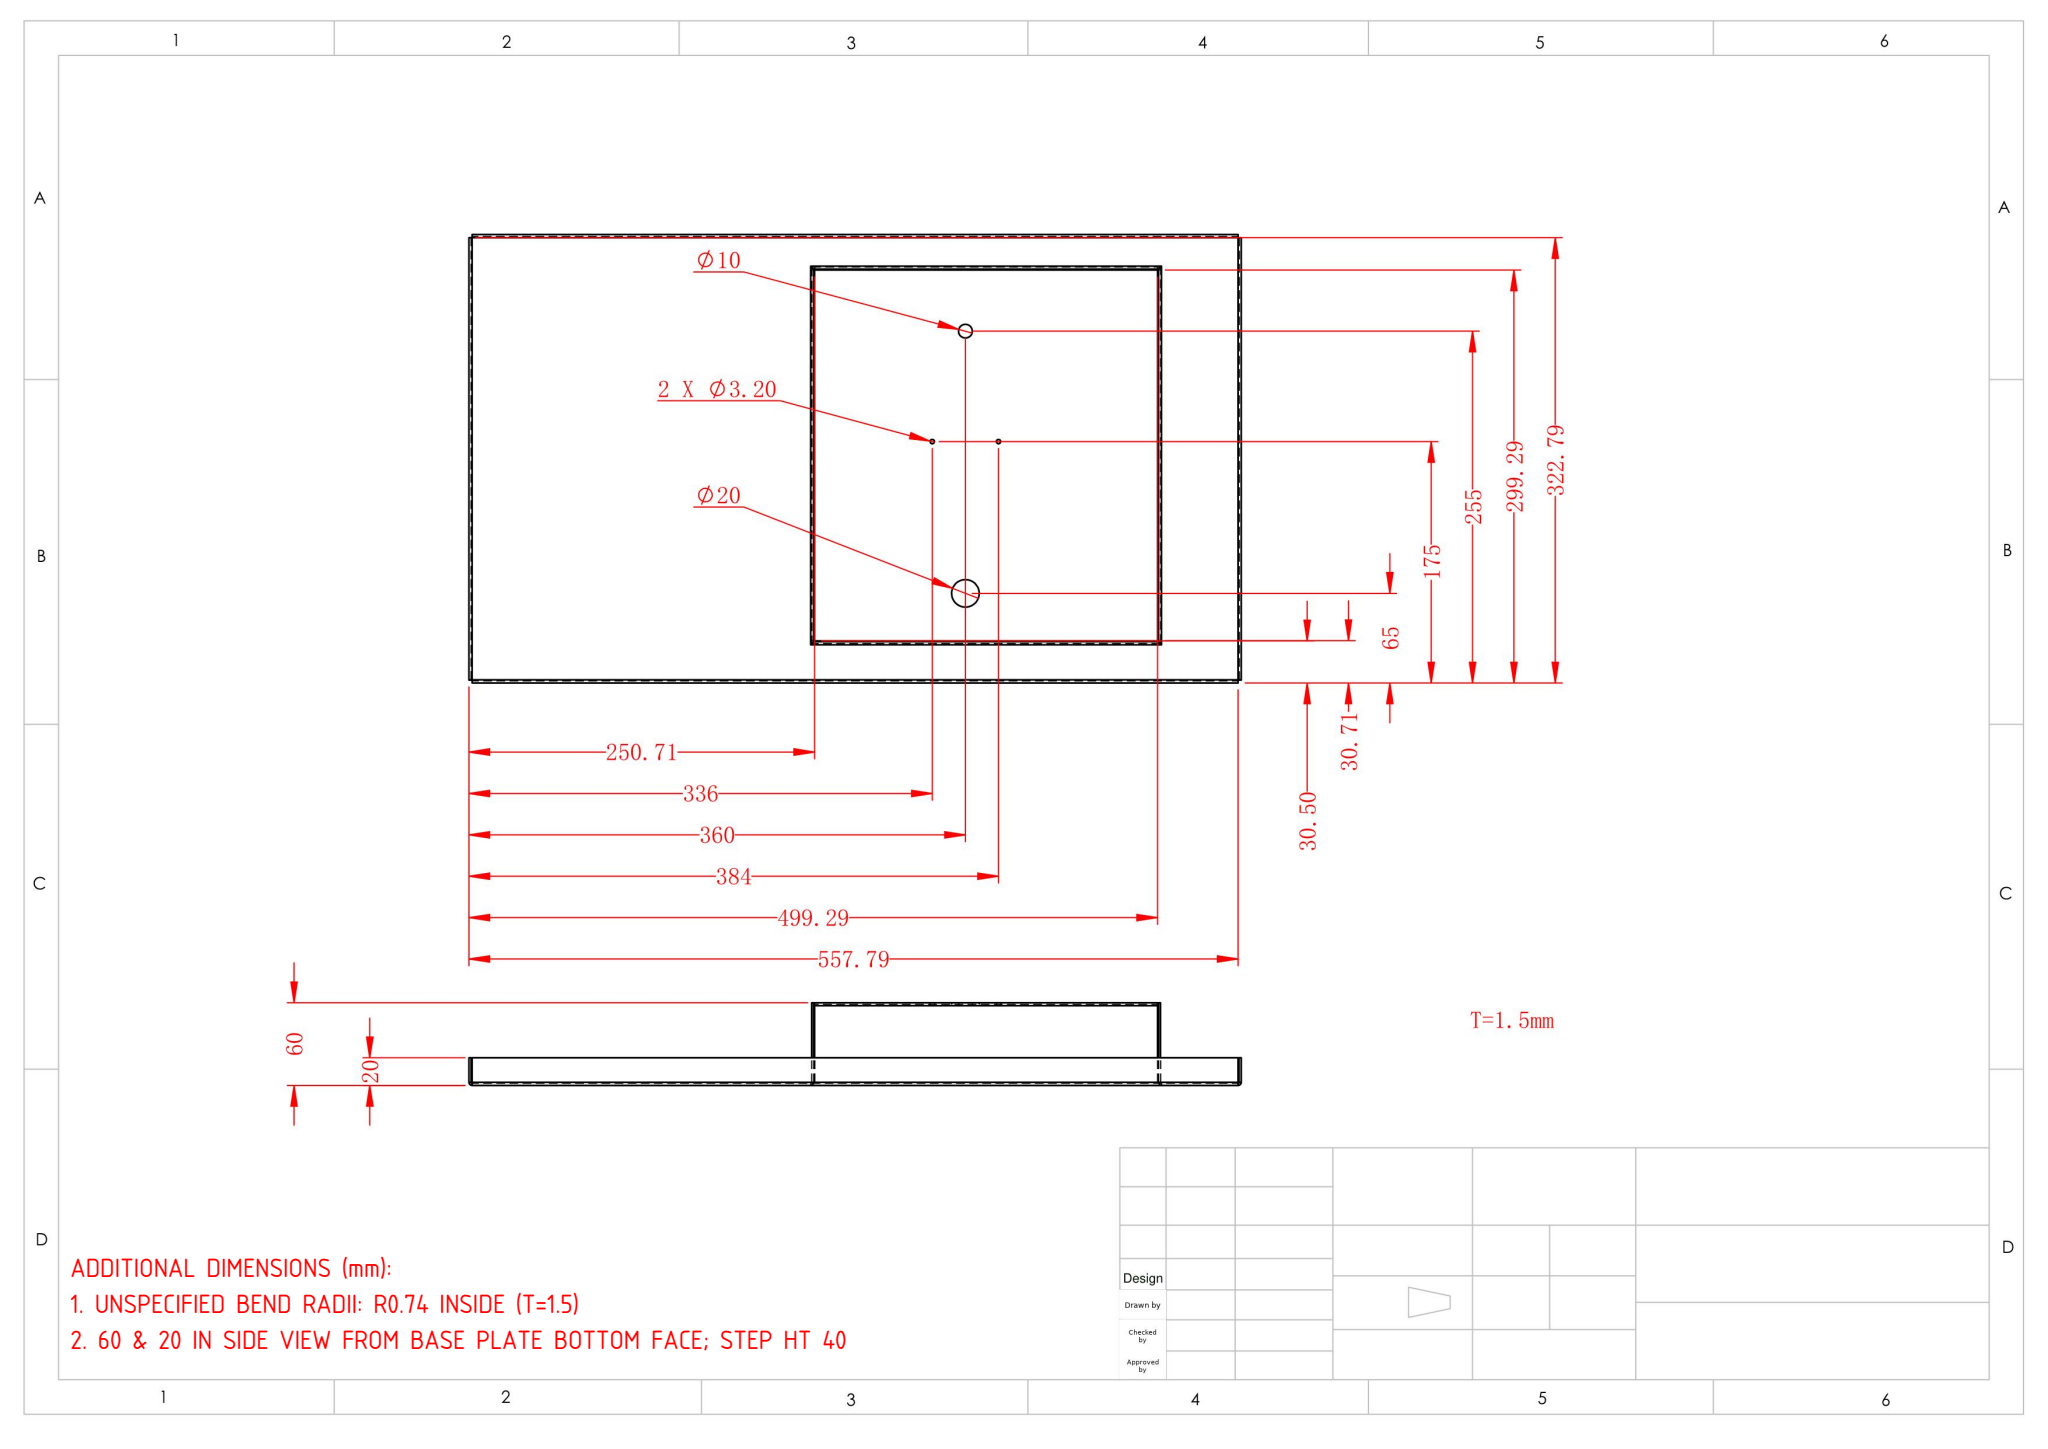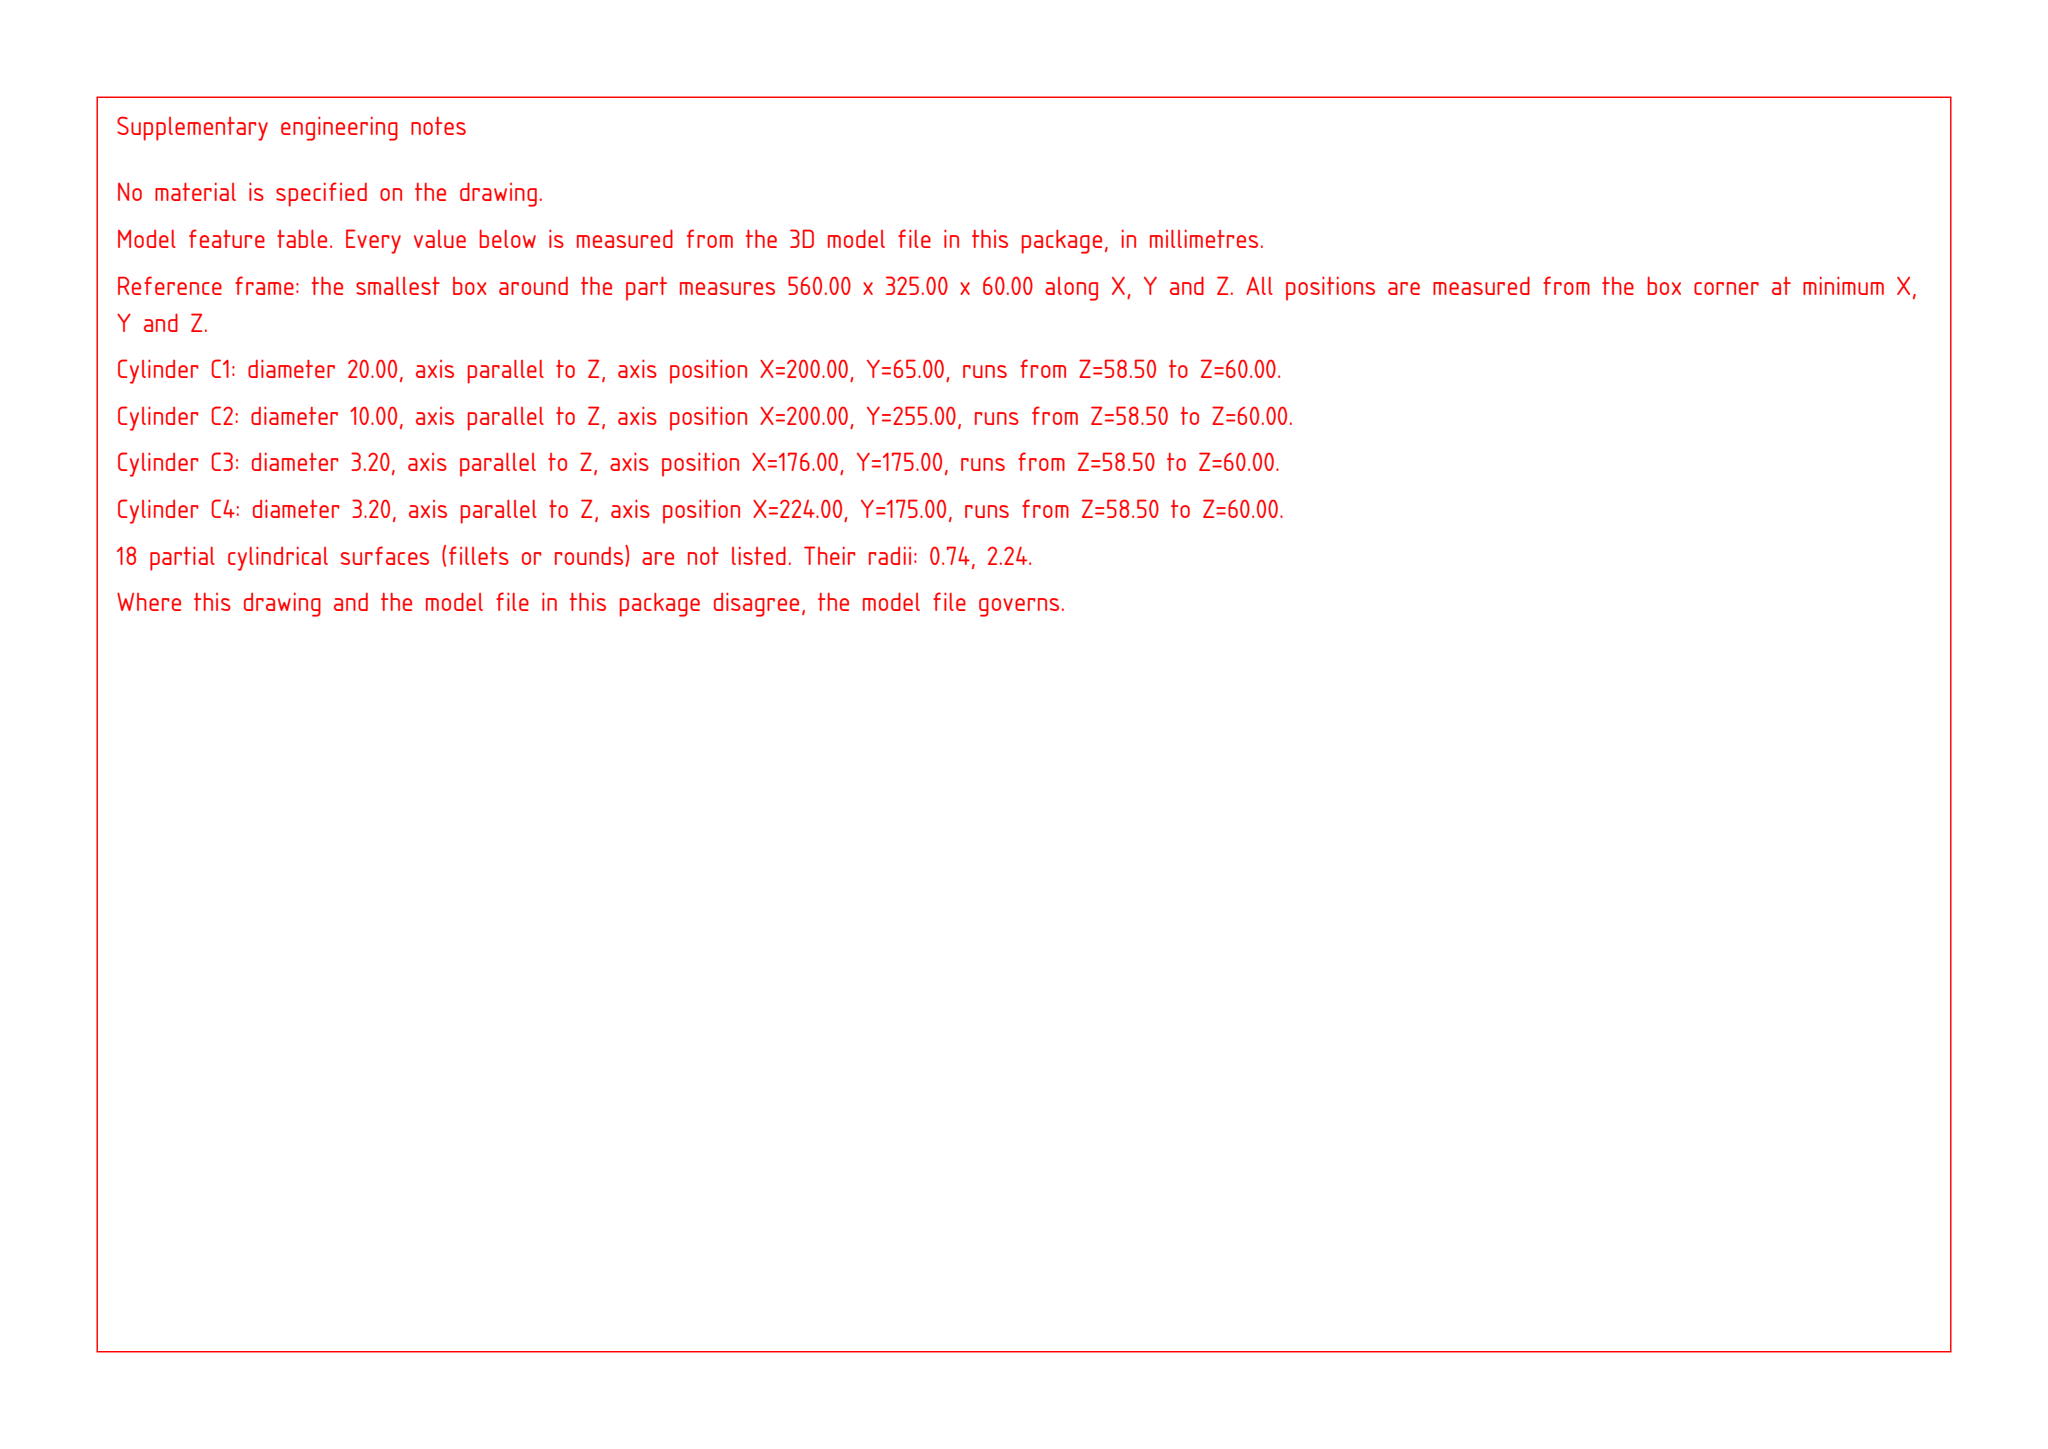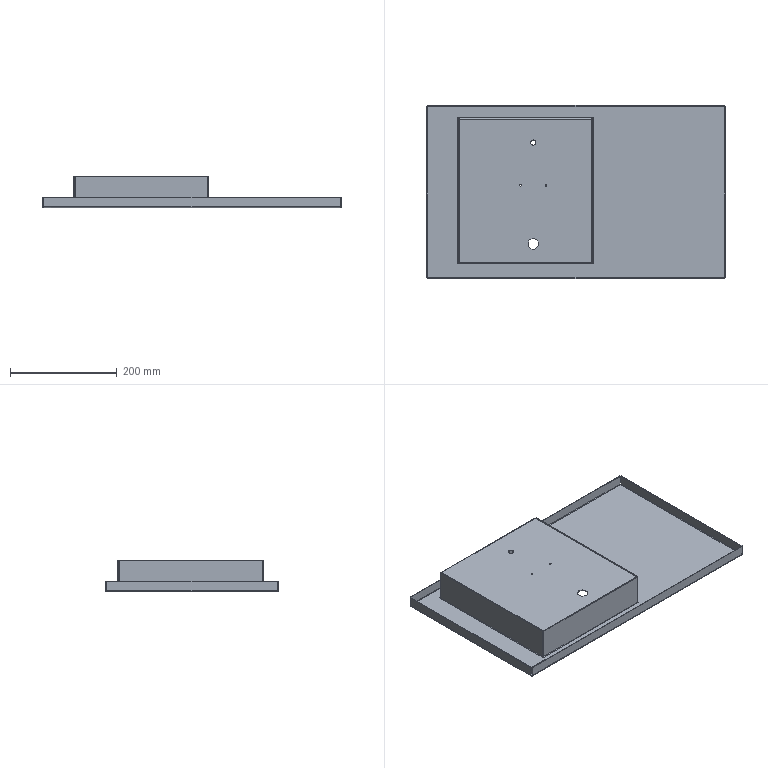Part | SolidWorks | mm | 1 solid | 90 faces | box 560 x 325 x 60 mm | volume 408076 mm3 | plane 48 | cylinder 26 | spline 16 | commonest cylinder face diameters 4.473 x9 1.473 x9 3.2 x4 10 x2 20 x2